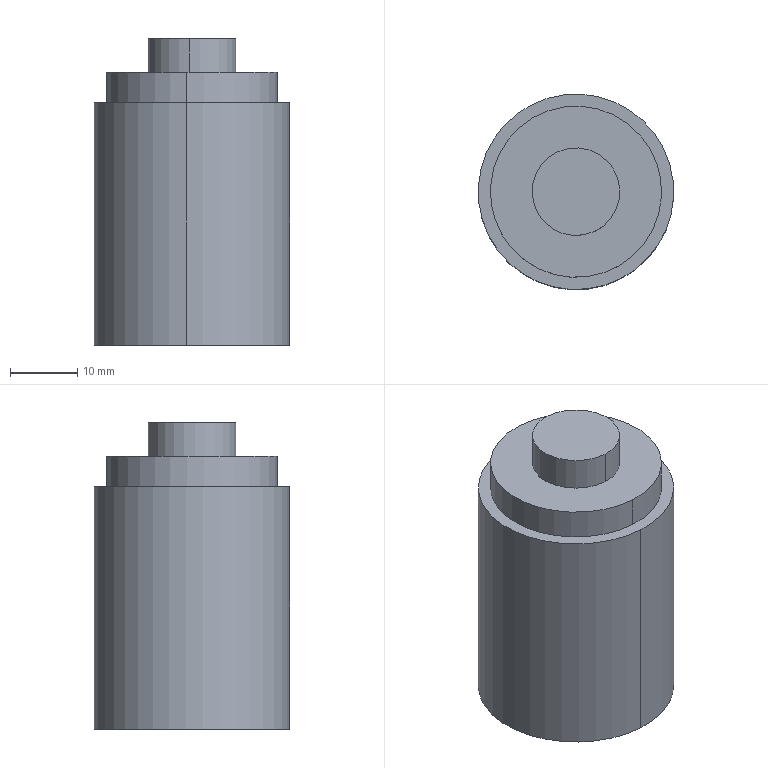Component | SolidWorks | Lens-2 | 1 solid | 13 faces | box 29 x 29 x 45.5 mm | volume 24719 mm3 | cylinder 8 | plane 5 | commonest cylinder face diameters 27 x2 13 x2 25.4 x2 29 x2 | material S45C
build123d program:
from build123d import *

# Parameters (mm, degrees)
SKETCH1_R           = 14.5
BOSS_EXTRUDE1_DEPTH = 36
SKETCH2_R           = 12.7
BOSS_EXTRUDE2_DEPTH = 4.5
SKETCH3_R           = 6.5
BOSS_EXTRUDE3_DEPTH = 5
SKETCH4_R           = 13.5
CUT_EXTRUDE1_DEPTH  = 3.5


with BuildPart() as part:
    # Sketch1 → Boss-Extrude1 (new body)
    with BuildSketch(Plane(origin=(0, 0, 0), x_dir=(1, 0, 0), z_dir=(0, 1, 0))):
        with Locations(Location((0, 0, 0), (0, 0, 270))):
            Circle(SKETCH1_R)
    extrude(amount=BOSS_EXTRUDE1_DEPTH)

    # Sketch2 → Boss-Extrude2 (add)
    with BuildSketch(Plane(origin=(0, 36, 0), x_dir=(1, 0, 0), z_dir=(0, 1, 0))):
        with Locations(Location((0, 0, 0), (0, 0, 270))):
            Circle(SKETCH2_R)
    extrude(amount=BOSS_EXTRUDE2_DEPTH)

    # Sketch3 → Boss-Extrude3 (add)
    with BuildSketch(Plane(origin=(0, 40.5, 0), x_dir=(1, 0, 0), z_dir=(0, 1, 0))):
        with Locations(Location((0, 0, 0), (0, 0, 270))):
            Circle(SKETCH3_R)
    extrude(amount=BOSS_EXTRUDE3_DEPTH)

    # Sketch4 → Cut-Extrude1 (cut)
    with BuildSketch(Plane.XZ):
        with Locations(Location((0, 0, 0), (0, 0, 270))):
            Circle(SKETCH4_R)
    extrude(amount=-CUT_EXTRUDE1_DEPTH, mode=Mode.SUBTRACT)


solid = part.part

# Placed as in the assembly
solid = solid.moved(Location((541.864, 441.164, 979.886), (90, 0, 0)))
STEP:
#1=COLOUR_RGB('',0.7922,0.8196,0.9333);
#2=FILL_AREA_STYLE_COLOUR('',#1);
#3=FILL_AREA_STYLE('',(#2));
#4=SURFACE_STYLE_FILL_AREA(#3);
#5=SURFACE_SIDE_STYLE('',(#4));
#6=SURFACE_STYLE_USAGE(.BOTH.,#5);
#7=PRESENTATION_STYLE_ASSIGNMENT((#6));
#8=CARTESIAN_POINT('',(21.302,16.838,38.716));
#9=VERTEX_POINT('',#8);
#10=CARTESIAN_POINT('',(21.365,17.899,38.716));
#11=VERTEX_POINT('',#10);
#12=CARTESIAN_POINT('',(21.333,17.369,38.716));
#13=DIRECTION('',(-0.,0.,-1.));
#14=DIRECTION('',(0.05929,0.9982,0.));
#15=AXIS2_PLACEMENT_3D('',#12,#13,#14);
#16=CIRCLE('',#15,0.5315);
#17=EDGE_CURVE('',#9,#11,#16,.T.);
#18=ORIENTED_EDGE('',*,*,#17,.F.);
#19=CARTESIAN_POINT('',(21.302,16.838,38.578));
#20=VERTEX_POINT('',#19);
#21=CARTESIAN_POINT('',(21.302,16.838,38.716));
#22=DIRECTION('',(-0.,0.,-1.));
#23=VECTOR('',#22,39.37);
#24=LINE('',#21,#23);
#25=EDGE_CURVE('',#9,#20,#24,.T.);
#26=ORIENTED_EDGE('',*,*,#25,.T.);
#27=CARTESIAN_POINT('',(21.365,17.899,38.578));
#28=VERTEX_POINT('',#27);
#29=CARTESIAN_POINT('',(21.333,17.369,38.578));
#30=DIRECTION('',(-0.,0.,-1.));
#31=DIRECTION('',(0.05929,0.9982,0.));
#32=AXIS2_PLACEMENT_3D('',#29,#30,#31);
#33=CIRCLE('',#32,0.5315);
#34=EDGE_CURVE('',#20,#28,#33,.T.);
#35=ORIENTED_EDGE('',*,*,#34,.T.);
#36=CARTESIAN_POINT('',(21.365,17.899,38.716));
#37=DIRECTION('',(-0.,0.,-1.));
#38=VECTOR('',#37,39.37);
#39=LINE('',#36,#38);
#40=EDGE_CURVE('',#11,#28,#39,.T.);
#41=ORIENTED_EDGE('',*,*,#40,.F.);
#42=EDGE_LOOP('',(#18,#26,#35,#41));
#43=FACE_OUTER_BOUND('',#42,.T.);
#44=CARTESIAN_POINT('',(21.333,17.369,38.716));
#45=DIRECTION('',(-0.,0.,-1.));
#46=DIRECTION('',(0.05929,0.9982,0.));
#47=AXIS2_PLACEMENT_3D('',#44,#45,#46);
#48=CYLINDRICAL_SURFACE('',#47,0.5315);
#49=ADVANCED_FACE('',(#43),#48,.F.);
#50=CARTESIAN_POINT('',(21.318,17.113,40.37));
#51=VERTEX_POINT('',#50);
#52=CARTESIAN_POINT('',(21.348,17.624,40.37));
#53=VERTEX_POINT('',#52);
#54=CARTESIAN_POINT('',(21.333,17.369,40.37));
#55=DIRECTION('',(0.,-0.,1.));
#56=DIRECTION('',(-0.05929,-0.9982,0.));
#57=AXIS2_PLACEMENT_3D('',#54,#55,#56);
#58=CIRCLE('',#57,0.2559);
#59=EDGE_CURVE('',#51,#53,#58,.T.);
#60=ORIENTED_EDGE('',*,*,#59,.F.);
#61=CARTESIAN_POINT('',(21.318,17.113,40.173));
#62=VERTEX_POINT('',#61);
#63=CARTESIAN_POINT('',(21.318,17.113,40.37));
#64=DIRECTION('',(-0.,0.,-1.));
#65=VECTOR('',#64,39.37);
#66=LINE('',#63,#65);
#67=EDGE_CURVE('',#51,#62,#66,.T.);
#68=ORIENTED_EDGE('',*,*,#67,.T.);
#69=CARTESIAN_POINT('',(21.348,17.624,40.173));
#70=VERTEX_POINT('',#69);
#71=CARTESIAN_POINT('',(21.333,17.369,40.173));
#72=DIRECTION('',(0.,-0.,1.));
#73=DIRECTION('',(-0.05929,-0.9982,0.));
#74=AXIS2_PLACEMENT_3D('',#71,#72,#73);
#75=CIRCLE('',#74,0.2559);
#76=EDGE_CURVE('',#62,#70,#75,.T.);
#77=ORIENTED_EDGE('',*,*,#76,.T.);
#78=CARTESIAN_POINT('',(21.348,17.624,40.37));
#79=DIRECTION('',(-0.,0.,-1.));
#80=VECTOR('',#79,39.37);
#81=LINE('',#78,#80);
#82=EDGE_CURVE('',#53,#70,#81,.T.);
#83=ORIENTED_EDGE('',*,*,#82,.F.);
#84=EDGE_LOOP('',(#60,#68,#77,#83));
#85=FACE_OUTER_BOUND('',#84,.T.);
#86=CARTESIAN_POINT('',(21.333,17.369,40.37));
#87=DIRECTION('',(-0.,0.,-1.));
#88=DIRECTION('',(0.05929,0.9982,0.));
#89=AXIS2_PLACEMENT_3D('',#86,#87,#88);
#90=CYLINDRICAL_SURFACE('',#89,0.2559);
#91=ADVANCED_FACE('',(#85),#90,.T.);
#92=CARTESIAN_POINT('',(21.304,16.87,40.173));
#93=VERTEX_POINT('',#92);
#94=CARTESIAN_POINT('',(21.363,17.868,40.173));
#95=VERTEX_POINT('',#94);
#96=CARTESIAN_POINT('',(21.333,17.369,40.173));
#97=DIRECTION('',(0.,-0.,1.));
#98=DIRECTION('',(-0.05929,-0.9982,0.));
#99=AXIS2_PLACEMENT_3D('',#96,#97,#98);
#100=CIRCLE('',#99,0.5);
#101=EDGE_CURVE('',#93,#95,#100,.T.);
#102=ORIENTED_EDGE('',*,*,#101,.F.);
#103=CARTESIAN_POINT('',(21.304,16.87,39.996));
#104=VERTEX_POINT('',#103);
#105=CARTESIAN_POINT('',(21.304,16.87,40.173));
#106=DIRECTION('',(-0.,0.,-1.));
#107=VECTOR('',#106,39.37);
#108=LINE('',#105,#107);
#109=EDGE_CURVE('',#93,#104,#108,.T.);
#110=ORIENTED_EDGE('',*,*,#109,.T.);
#111=CARTESIAN_POINT('',(21.363,17.868,39.996));
#112=VERTEX_POINT('',#111);
#113=CARTESIAN_POINT('',(21.333,17.369,39.996));
#114=DIRECTION('',(0.,-0.,1.));
#115=DIRECTION('',(-0.05929,-0.9982,0.));
#116=AXIS2_PLACEMENT_3D('',#113,#114,#115);
#117=CIRCLE('',#116,0.5);
#118=EDGE_CURVE('',#104,#112,#117,.T.);
#119=ORIENTED_EDGE('',*,*,#118,.T.);
#120=CARTESIAN_POINT('',(21.363,17.868,40.173));
#121=DIRECTION('',(-0.,0.,-1.));
#122=VECTOR('',#121,39.37);
#123=LINE('',#120,#122);
#124=EDGE_CURVE('',#95,#112,#123,.T.);
#125=ORIENTED_EDGE('',*,*,#124,.F.);
#126=EDGE_LOOP('',(#102,#110,#119,#125));
#127=FACE_OUTER_BOUND('',#126,.T.);
#128=CARTESIAN_POINT('',(21.333,17.369,40.173));
#129=DIRECTION('',(-0.,0.,-1.));
#130=DIRECTION('',(0.05929,0.9982,0.));
#131=AXIS2_PLACEMENT_3D('',#128,#129,#130);
#132=CYLINDRICAL_SURFACE('',#131,0.5);
#133=ADVANCED_FACE('',(#127),#132,.T.);
#134=CARTESIAN_POINT('',(21.299,16.799,39.996));
#135=VERTEX_POINT('',#134);
#136=CARTESIAN_POINT('',(21.367,17.939,39.996));
#137=VERTEX_POINT('',#136);
#138=CARTESIAN_POINT('',(21.333,17.369,39.996));
#139=DIRECTION('',(0.,-0.,1.));
#140=DIRECTION('',(-0.05929,-0.9982,0.));
#141=AXIS2_PLACEMENT_3D('',#138,#139,#140);
#142=CIRCLE('',#141,0.5709);
#143=EDGE_CURVE('',#135,#137,#142,.T.);
#144=ORIENTED_EDGE('',*,*,#143,.F.);
#145=CARTESIAN_POINT('',(21.299,16.799,38.578));
#146=VERTEX_POINT('',#145);
#147=CARTESIAN_POINT('',(21.299,16.799,39.996));
#148=DIRECTION('',(-0.,0.,-1.));
#149=VECTOR('',#148,39.37);
#150=LINE('',#147,#149);
#151=EDGE_CURVE('',#135,#146,#150,.T.);
#152=ORIENTED_EDGE('',*,*,#151,.T.);
#153=CARTESIAN_POINT('',(21.367,17.939,38.578));
#154=VERTEX_POINT('',#153);
#155=CARTESIAN_POINT('',(21.333,17.369,38.578));
#156=DIRECTION('',(0.,-0.,1.));
#157=DIRECTION('',(-0.05929,-0.9982,0.));
#158=AXIS2_PLACEMENT_3D('',#155,#156,#157);
#159=CIRCLE('',#158,0.5709);
#160=EDGE_CURVE('',#146,#154,#159,.T.);
#161=ORIENTED_EDGE('',*,*,#160,.T.);
#162=CARTESIAN_POINT('',(21.367,17.939,39.996));
#163=DIRECTION('',(-0.,0.,-1.));
#164=VECTOR('',#163,39.37);
#165=LINE('',#162,#164);
#166=EDGE_CURVE('',#137,#154,#165,.T.);
#167=ORIENTED_EDGE('',*,*,#166,.F.);
#168=EDGE_LOOP('',(#144,#152,#161,#167));
#169=FACE_OUTER_BOUND('',#168,.T.);
#170=CARTESIAN_POINT('',(21.333,17.369,39.996));
#171=DIRECTION('',(-0.,0.,-1.));
#172=DIRECTION('',(0.05929,0.9982,0.));
#173=AXIS2_PLACEMENT_3D('',#170,#171,#172);
#174=CYLINDRICAL_SURFACE('',#173,0.5709);
#175=ADVANCED_FACE('',(#169),#174,.T.);
#176=ORIENTED_EDGE('',*,*,#151,.F.);
#177=CARTESIAN_POINT('',(21.333,17.369,39.996));
#178=DIRECTION('',(0.,-0.,1.));
#179=DIRECTION('',(-0.05929,-0.9982,0.));
#180=AXIS2_PLACEMENT_3D('',#177,#178,#179);
#181=CIRCLE('',#180,0.5709);
#182=EDGE_CURVE('',#137,#135,#181,.T.);
#183=ORIENTED_EDGE('',*,*,#182,.F.);
#184=ORIENTED_EDGE('',*,*,#166,.T.);
#185=CARTESIAN_POINT('',(21.333,17.369,38.578));
#186=DIRECTION('',(0.,-0.,1.));
#187=DIRECTION('',(-0.05929,-0.9982,0.));
#188=AXIS2_PLACEMENT_3D('',#185,#186,#187);
#189=CIRCLE('',#188,0.5709);
#190=EDGE_CURVE('',#154,#146,#189,.T.);
#191=ORIENTED_EDGE('',*,*,#190,.T.);
#192=EDGE_LOOP('',(#176,#183,#184,#191));
#193=FACE_OUTER_BOUND('',#192,.T.);
#194=CARTESIAN_POINT('',(21.333,17.369,39.996));
#195=DIRECTION('',(-0.,0.,-1.));
#196=DIRECTION('',(0.05929,0.9982,0.));
#197=AXIS2_PLACEMENT_3D('',#194,#195,#196);
#198=CYLINDRICAL_SURFACE('',#197,0.5709);
#199=ADVANCED_FACE('',(#193),#198,.T.);
#200=CARTESIAN_POINT('',(21.333,17.369,39.996));
#201=DIRECTION('',(0.,-0.,1.));
#202=DIRECTION('',(-0.05929,-0.9982,0.));
#203=AXIS2_PLACEMENT_3D('',#200,#201,#202);
#204=CIRCLE('',#203,0.5);
#205=EDGE_CURVE('',#112,#104,#204,.T.);
#206=ORIENTED_EDGE('',*,*,#205,.F.);
#207=ORIENTED_EDGE('',*,*,#118,.F.);
#208=EDGE_LOOP('',(#206,#207));
#209=FACE_BOUND('',#208,.T.);
#210=ORIENTED_EDGE('',*,*,#182,.T.);
#211=ORIENTED_EDGE('',*,*,#143,.T.);
#212=EDGE_LOOP('',(#210,#211));
#213=FACE_OUTER_BOUND('',#212,.T.);
#214=CARTESIAN_POINT('',(21.333,17.369,39.996));
#215=DIRECTION('',(0.,-0.,1.));
#216=DIRECTION('',(-0.05929,-0.9982,-0.));
#217=AXIS2_PLACEMENT_3D('',#214,#215,#216);
#218=PLANE('',#217);
#219=ADVANCED_FACE('',(#209,#213),#218,.T.);
#220=CARTESIAN_POINT('',(21.333,17.369,38.578));
#221=DIRECTION('',(-0.,0.,-1.));
#222=DIRECTION('',(0.05929,0.9982,0.));
#223=AXIS2_PLACEMENT_3D('',#220,#221,#222);
#224=CIRCLE('',#223,0.5315);
#225=EDGE_CURVE('',#28,#20,#224,.T.);
#226=ORIENTED_EDGE('',*,*,#225,.F.);
#227=ORIENTED_EDGE('',*,*,#34,.F.);
#228=EDGE_LOOP('',(#226,#227));
#229=FACE_BOUND('',#228,.T.);
#230=ORIENTED_EDGE('',*,*,#190,.F.);
#231=ORIENTED_EDGE('',*,*,#160,.F.);
#232=EDGE_LOOP('',(#230,#231));
#233=FACE_OUTER_BOUND('',#232,.T.);
#234=CARTESIAN_POINT('',(21.333,17.369,38.578));
#235=DIRECTION('',(0.,-0.,1.));
#236=DIRECTION('',(-0.05929,-0.9982,-0.));
#237=AXIS2_PLACEMENT_3D('',#234,#235,#236);
#238=PLANE('',#237);
#239=ADVANCED_FACE('',(#229,#233),#238,.F.);
#240=ORIENTED_EDGE('',*,*,#109,.F.);
#241=CARTESIAN_POINT('',(21.333,17.369,40.173));
#242=DIRECTION('',(0.,-0.,1.));
#243=DIRECTION('',(-0.05929,-0.9982,0.));
#244=AXIS2_PLACEMENT_3D('',#241,#242,#243);
#245=CIRCLE('',#244,0.5);
#246=EDGE_CURVE('',#95,#93,#245,.T.);
#247=ORIENTED_EDGE('',*,*,#246,.F.);
#248=ORIENTED_EDGE('',*,*,#124,.T.);
#249=ORIENTED_EDGE('',*,*,#205,.T.);
#250=EDGE_LOOP('',(#240,#247,#248,#249));
#251=FACE_OUTER_BOUND('',#250,.T.);
#252=CARTESIAN_POINT('',(21.333,17.369,40.173));
#253=DIRECTION('',(-0.,0.,-1.));
#254=DIRECTION('',(0.05929,0.9982,0.));
#255=AXIS2_PLACEMENT_3D('',#252,#253,#254);
#256=CYLINDRICAL_SURFACE('',#255,0.5);
#257=ADVANCED_FACE('',(#251),#256,.T.);
#258=CARTESIAN_POINT('',(21.333,17.369,40.173));
#259=DIRECTION('',(0.,-0.,1.));
#260=DIRECTION('',(-0.05929,-0.9982,0.));
#261=AXIS2_PLACEMENT_3D('',#258,#259,#260);
#262=CIRCLE('',#261,0.2559);
#263=EDGE_CURVE('',#70,#62,#262,.T.);
#264=ORIENTED_EDGE('',*,*,#263,.F.);
#265=ORIENTED_EDGE('',*,*,#76,.F.);
#266=EDGE_LOOP('',(#264,#265));
#267=FACE_BOUND('',#266,.T.);
#268=ORIENTED_EDGE('',*,*,#246,.T.);
#269=ORIENTED_EDGE('',*,*,#101,.T.);
#270=EDGE_LOOP('',(#268,#269));
#271=FACE_OUTER_BOUND('',#270,.T.);
#272=CARTESIAN_POINT('',(21.333,17.369,40.173));
#273=DIRECTION('',(0.,-0.,1.));
#274=DIRECTION('',(-0.05929,-0.9982,-0.));
#275=AXIS2_PLACEMENT_3D('',#272,#273,#274);
#276=PLANE('',#275);
#277=ADVANCED_FACE('',(#267,#271),#276,.T.);
#278=ORIENTED_EDGE('',*,*,#67,.F.);
#279=CARTESIAN_POINT('',(21.333,17.369,40.37));
#280=DIRECTION('',(0.,-0.,1.));
#281=DIRECTION('',(-0.05929,-0.9982,0.));
#282=AXIS2_PLACEMENT_3D('',#279,#280,#281);
#283=CIRCLE('',#282,0.2559);
#284=EDGE_CURVE('',#53,#51,#283,.T.);
#285=ORIENTED_EDGE('',*,*,#284,.F.);
#286=ORIENTED_EDGE('',*,*,#82,.T.);
#287=ORIENTED_EDGE('',*,*,#263,.T.);
#288=EDGE_LOOP('',(#278,#285,#286,#287));
#289=FACE_OUTER_BOUND('',#288,.T.);
#290=CARTESIAN_POINT('',(21.333,17.369,40.37));
#291=DIRECTION('',(-0.,0.,-1.));
#292=DIRECTION('',(0.05929,0.9982,0.));
#293=AXIS2_PLACEMENT_3D('',#290,#291,#292);
#294=CYLINDRICAL_SURFACE('',#293,0.2559);
#295=ADVANCED_FACE('',(#289),#294,.T.);
#296=ORIENTED_EDGE('',*,*,#284,.T.);
#297=ORIENTED_EDGE('',*,*,#59,.T.);
#298=EDGE_LOOP('',(#296,#297));
#299=FACE_OUTER_BOUND('',#298,.T.);
#300=CARTESIAN_POINT('',(21.333,17.369,40.37));
#301=DIRECTION('',(0.,-0.,1.));
#302=DIRECTION('',(-0.05929,-0.9982,-0.));
#303=AXIS2_PLACEMENT_3D('',#300,#301,#302);
#304=PLANE('',#303);
#305=ADVANCED_FACE('',(#299),#304,.T.);
#306=ORIENTED_EDGE('',*,*,#25,.F.);
#307=CARTESIAN_POINT('',(21.333,17.369,38.716));
#308=DIRECTION('',(-0.,0.,-1.));
#309=DIRECTION('',(0.05929,0.9982,0.));
#310=AXIS2_PLACEMENT_3D('',#307,#308,#309);
#311=CIRCLE('',#310,0.5315);
#312=EDGE_CURVE('',#11,#9,#311,.T.);
#313=ORIENTED_EDGE('',*,*,#312,.F.);
#314=ORIENTED_EDGE('',*,*,#40,.T.);
#315=ORIENTED_EDGE('',*,*,#225,.T.);
#316=EDGE_LOOP('',(#306,#313,#314,#315));
#317=FACE_OUTER_BOUND('',#316,.T.);
#318=CARTESIAN_POINT('',(21.333,17.369,38.716));
#319=DIRECTION('',(-0.,0.,-1.));
#320=DIRECTION('',(0.05929,0.9982,0.));
#321=AXIS2_PLACEMENT_3D('',#318,#319,#320);
#322=CYLINDRICAL_SURFACE('',#321,0.5315);
#323=ADVANCED_FACE('',(#317),#322,.F.);
#324=ORIENTED_EDGE('',*,*,#312,.T.);
#325=ORIENTED_EDGE('',*,*,#17,.T.);
#326=EDGE_LOOP('',(#324,#325));
#327=FACE_OUTER_BOUND('',#326,.T.);
#328=CARTESIAN_POINT('',(21.333,17.369,38.716));
#329=DIRECTION('',(-0.,0.,-1.));
#330=DIRECTION('',(0.05929,0.9982,0.));
#331=AXIS2_PLACEMENT_3D('',#328,#329,#330);
#332=PLANE('',#331);
#333=ADVANCED_FACE('',(#327),#332,.T.);
#334=CLOSED_SHELL('',(#49,#91,#133,#175,#199,#219,#239,#257,#277,#295,#305,#323,#333));
#335=MANIFOLD_SOLID_BREP('',#334);
#336=STYLED_ITEM('',(#7),#335);
#337=(LENGTH_UNIT()NAMED_UNIT(*)SI_UNIT($,.METRE.));
#338=LENGTH_MEASURE_WITH_UNIT(LENGTH_MEASURE(0.0254),#337);
#339=DIMENSIONAL_EXPONENTS(1.,0.,0.,0.,0.,0.,0.);
#340=(CONVERSION_BASED_UNIT('',#338)LENGTH_UNIT()NAMED_UNIT(#339));
#341=UNCERTAINTY_MEASURE_WITH_UNIT(LENGTH_MEASURE(0.00001),#340,'','');
#342=(NAMED_UNIT(*)PLANE_ANGLE_UNIT()SI_UNIT($,.RADIAN.));
#343=(NAMED_UNIT(*)SI_UNIT($,.STERADIAN.)SOLID_ANGLE_UNIT());
#344=(GEOMETRIC_REPRESENTATION_CONTEXT(3)GLOBAL_UNCERTAINTY_ASSIGNED_CONTEXT((#341))GLOBAL_UNIT_ASSIGNED_CONTEXT((#340,#342,#343))REPRESENTATION_CONTEXT('',''));
#345=MECHANICAL_DESIGN_GEOMETRIC_PRESENTATION_REPRESENTATION('',(#336),#344);
#346=PRESENTATION_LAYER_ASSIGNMENT('','',(#336));
#347=CARTESIAN_POINT('',(0.,0.,0.));
#348=DIRECTION('',(0.,0.,1.));
#349=DIRECTION('',(1.,0.,0.));
#350=AXIS2_PLACEMENT_3D('',#347,#348,#349);
#351=(LENGTH_UNIT()NAMED_UNIT(*)SI_UNIT($,.METRE.));
#352=LENGTH_MEASURE_WITH_UNIT(LENGTH_MEASURE(0.0254),#351);
#353=DIMENSIONAL_EXPONENTS(1.,0.,0.,0.,0.,0.,0.);
#354=(CONVERSION_BASED_UNIT('',#352)LENGTH_UNIT()NAMED_UNIT(#353));
#355=UNCERTAINTY_MEASURE_WITH_UNIT(LENGTH_MEASURE(0.00001),#354,'','');
#356=(NAMED_UNIT(*)PLANE_ANGLE_UNIT()SI_UNIT($,.RADIAN.));
#357=(NAMED_UNIT(*)SI_UNIT($,.STERADIAN.)SOLID_ANGLE_UNIT());
#358=(GEOMETRIC_REPRESENTATION_CONTEXT(3)GLOBAL_UNCERTAINTY_ASSIGNED_CONTEXT((#355))GLOBAL_UNIT_ASSIGNED_CONTEXT((#354,#356,#357))REPRESENTATION_CONTEXT('',''));
#359=ADVANCED_BREP_SHAPE_REPRESENTATION('',(#335,#350),#358);